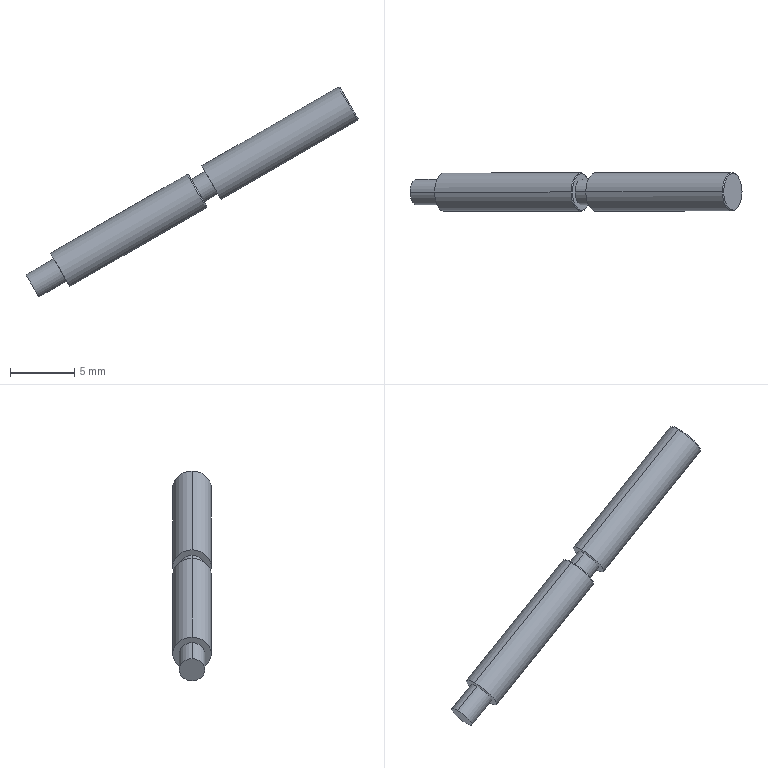Component | SolidWorks | SliderScrew1-1 | 1 solid | 17 faces | box 25.89 x 3 x 16.38 mm | volume 187 mm3 | cylinder 8 | plane 5 | cone 4 | commonest cylinder face diameters 2 x4 3 x4
build123d program:
from build123d import *

# Parameters (mm, degrees)
SKETCH1_R           = 1.5
BOSS_EXTRUDE1_DEPTH = 13
CHAMFER1_SIZE       = 0.08
SKETCH2_R           = 1.5
SKETCH2_R_2         = 1
CUT_EXTRUDE1_DEPTH  = 0.625
CHAMFER2_SIZE       = 0.08
BOSS_EXTRUDE2_START = 2.5
SKETCH3_R           = 1
BOSS_EXTRUDE2_DEPTH = 2.5


with BuildPart() as part:
    # Sketch1 → Boss-Extrude1 (new, symmetric)
    with BuildSketch(Plane(origin=(0, 0, 0), x_dir=(0, 0, -1), z_dir=(1, 0, 0))):
        with Locations(Location((0, 0, 0), (0, 0, 180))):
            Circle(SKETCH1_R)
    extrude(amount=BOSS_EXTRUDE1_DEPTH, both=True)

    # Chamfer1
    chamfer1_edges = [part.edges().sort_by_distance(p)[0] for p in [
        (13, 0, -1.5),
    ]]
    chamfer(chamfer1_edges, length=CHAMFER1_SIZE)

    # Sketch2 → Cut-Extrude1 (cut, symmetric)
    with BuildSketch(Plane(origin=(0, 0, 0), x_dir=(0, 0, -1), z_dir=(1, 0, 0))):
        with Locations(Location((0, 0, 0), (0, 0, 180))):
            Circle(SKETCH2_R)
        Circle(SKETCH2_R_2, mode=Mode.SUBTRACT)
    extrude(amount=CUT_EXTRUDE1_DEPTH, both=True, mode=Mode.SUBTRACT)

    # Chamfer2
    chamfer2_edges = [part.edges().sort_by_distance(p)[0] for p in [
        (-0.625, 0, -1.5),
    ]]
    chamfer(chamfer2_edges, length=CHAMFER2_SIZE)

    # Sketch3 → Boss-Extrude2 (add)
    with BuildSketch(Plane.ZY.offset(13).offset(BOSS_EXTRUDE2_START)):
        with Locations(Location((0, 0, 0), (0, 0, 180))):
            Circle(SKETCH3_R)
    extrude(amount=-BOSS_EXTRUDE2_DEPTH)


solid = part.part

# Placed as in the assembly
solid = solid.moved(Location((-69.691, 19.006, 123.217), (-94.246, 2.447, -29.909)))
STEP:
#1=CARTESIAN_POINT('',(-3.292,0.7483,4.58));
#2=VERTEX_POINT('',#1);
#3=CARTESIAN_POINT('',(-3.253,0.7483,4.512));
#4=VERTEX_POINT('',#3);
#5=CARTESIAN_POINT('',(-3.272,0.7483,4.546));
#6=DIRECTION('',(-0.866,0.,-0.5));
#7=DIRECTION('',(-0.5,-0.00000096,0.866));
#8=AXIS2_PLACEMENT_3D('',#5,#6,#7);
#9=CIRCLE('',#8,0.03937);
#10=EDGE_CURVE('',#2,#4,#9,.T.);
#11=ORIENTED_EDGE('',*,*,#10,.F.);
#12=CARTESIAN_POINT('',(-3.207,0.7483,4.629));
#13=VERTEX_POINT('',#12);
#14=CARTESIAN_POINT('',(-3.292,0.7483,4.58));
#15=DIRECTION('',(0.866,-0.,0.5));
#16=VECTOR('',#15,39.37);
#17=LINE('',#14,#16);
#18=EDGE_CURVE('',#2,#13,#17,.T.);
#19=ORIENTED_EDGE('',*,*,#18,.T.);
#20=CARTESIAN_POINT('',(-3.167,0.7483,4.561));
#21=VERTEX_POINT('',#20);
#22=CARTESIAN_POINT('',(-3.187,0.7483,4.595));
#23=DIRECTION('',(-0.866,0.,-0.5));
#24=DIRECTION('',(-0.5,-0.00000096,0.866));
#25=AXIS2_PLACEMENT_3D('',#22,#23,#24);
#26=CIRCLE('',#25,0.03937);
#27=EDGE_CURVE('',#13,#21,#26,.T.);
#28=ORIENTED_EDGE('',*,*,#27,.T.);
#29=CARTESIAN_POINT('',(-3.253,0.7483,4.512));
#30=DIRECTION('',(0.866,-0.,0.5));
#31=VECTOR('',#30,39.37);
#32=LINE('',#29,#31);
#33=EDGE_CURVE('',#4,#21,#32,.T.);
#34=ORIENTED_EDGE('',*,*,#33,.F.);
#35=EDGE_LOOP('',(#11,#19,#28,#34));
#36=FACE_OUTER_BOUND('',#35,.T.);
#37=CARTESIAN_POINT('',(-3.272,0.7483,4.546));
#38=DIRECTION('',(0.866,-0.,0.5));
#39=DIRECTION('',(0.5,0.00000096,-0.866));
#40=AXIS2_PLACEMENT_3D('',#37,#38,#39);
#41=CYLINDRICAL_SURFACE('',#40,0.03937);
#42=ADVANCED_FACE('',(#36),#41,.T.);
#43=CARTESIAN_POINT('',(-2.737,0.7483,4.79));
#44=VERTEX_POINT('',#43);
#45=CARTESIAN_POINT('',(-2.793,0.7483,4.887));
#46=VERTEX_POINT('',#45);
#47=CARTESIAN_POINT('',(-2.765,0.7483,4.839));
#48=DIRECTION('',(0.866,-0.,0.5));
#49=DIRECTION('',(0.5,0.00000096,-0.866));
#50=AXIS2_PLACEMENT_3D('',#47,#48,#49);
#51=CIRCLE('',#50,0.05591);
#52=EDGE_CURVE('',#44,#46,#51,.T.);
#53=ORIENTED_EDGE('',*,*,#52,.F.);
#54=CARTESIAN_POINT('',(-2.738,0.7483,4.786));
#55=VERTEX_POINT('',#54);
#56=CARTESIAN_POINT('',(-2.737,0.7483,4.79));
#57=DIRECTION('',(-0.2588,0.00000068,-0.9659));
#58=VECTOR('',#57,39.37);
#59=LINE('',#56,#58);
#60=EDGE_CURVE('',#44,#55,#59,.T.);
#61=ORIENTED_EDGE('',*,*,#60,.T.);
#62=CARTESIAN_POINT('',(-2.797,0.7483,4.888));
#63=VERTEX_POINT('',#62);
#64=CARTESIAN_POINT('',(-2.768,0.7483,4.837));
#65=DIRECTION('',(-0.866,0.,-0.5));
#66=DIRECTION('',(0.5,0.00000096,-0.866));
#67=AXIS2_PLACEMENT_3D('',#64,#65,#66);
#68=CIRCLE('',#67,0.05906);
#69=EDGE_CURVE('',#63,#55,#68,.T.);
#70=ORIENTED_EDGE('',*,*,#69,.F.);
#71=CARTESIAN_POINT('',(-2.793,0.7483,4.887));
#72=DIRECTION('',(-0.9659,-0.00000068,0.2588));
#73=VECTOR('',#72,39.37);
#74=LINE('',#71,#73);
#75=EDGE_CURVE('',#46,#63,#74,.T.);
#76=ORIENTED_EDGE('',*,*,#75,.F.);
#77=EDGE_LOOP('',(#53,#61,#70,#76));
#78=FACE_OUTER_BOUND('',#77,.T.);
#79=CARTESIAN_POINT('',(-2.765,0.7483,4.839));
#80=DIRECTION('',(-0.866,0.,-0.5));
#81=DIRECTION('',(-0.5,-0.00000096,0.866));
#82=AXIS2_PLACEMENT_3D('',#79,#80,#81);
#83=CONICAL_SURFACE('',#82,0.05591,0.7854);
#84=ADVANCED_FACE('',(#78),#83,.T.);
#85=ORIENTED_EDGE('',*,*,#69,.T.);
#86=CARTESIAN_POINT('',(-3.157,0.7483,4.544));
#87=VERTEX_POINT('',#86);
#88=CARTESIAN_POINT('',(-2.271,0.7483,5.056));
#89=DIRECTION('',(-0.866,0.,-0.5));
#90=VECTOR('',#89,39.37);
#91=LINE('',#88,#90);
#92=EDGE_CURVE('',#55,#87,#91,.T.);
#93=ORIENTED_EDGE('',*,*,#92,.T.);
#94=CARTESIAN_POINT('',(-3.217,0.7483,4.646));
#95=VERTEX_POINT('',#94);
#96=CARTESIAN_POINT('',(-3.187,0.7483,4.595));
#97=DIRECTION('',(0.866,-0.,0.5));
#98=DIRECTION('',(0.5,0.00000096,-0.866));
#99=AXIS2_PLACEMENT_3D('',#96,#97,#98);
#100=CIRCLE('',#99,0.05906);
#101=EDGE_CURVE('',#87,#95,#100,.T.);
#102=ORIENTED_EDGE('',*,*,#101,.T.);
#103=CARTESIAN_POINT('',(-2.33,0.7483,5.158));
#104=DIRECTION('',(-0.866,0.,-0.5));
#105=VECTOR('',#104,39.37);
#106=LINE('',#103,#105);
#107=EDGE_CURVE('',#63,#95,#106,.T.);
#108=ORIENTED_EDGE('',*,*,#107,.F.);
#109=EDGE_LOOP('',(#85,#93,#102,#108));
#110=FACE_OUTER_BOUND('',#109,.T.);
#111=CARTESIAN_POINT('',(-2.301,0.7483,5.107));
#112=DIRECTION('',(-0.866,0.,-0.5));
#113=DIRECTION('',(-0.5,-0.00000096,0.866));
#114=AXIS2_PLACEMENT_3D('',#111,#112,#113);
#115=CYLINDRICAL_SURFACE('',#114,0.05906);
#116=ADVANCED_FACE('',(#110),#115,.T.);
#117=CARTESIAN_POINT('',(-2.745,0.7483,4.805));
#118=VERTEX_POINT('',#117);
#119=CARTESIAN_POINT('',(-2.785,0.7483,4.873));
#120=VERTEX_POINT('',#119);
#121=CARTESIAN_POINT('',(-2.765,0.7483,4.839));
#122=DIRECTION('',(0.866,-0.,0.5));
#123=DIRECTION('',(0.5,0.00000096,-0.866));
#124=AXIS2_PLACEMENT_3D('',#121,#122,#123);
#125=CIRCLE('',#124,0.03937);
#126=EDGE_CURVE('',#118,#120,#125,.T.);
#127=ORIENTED_EDGE('',*,*,#126,.T.);
#128=CARTESIAN_POINT('',(-2.742,0.7483,4.897));
#129=VERTEX_POINT('',#128);
#130=CARTESIAN_POINT('',(-2.785,0.7483,4.873));
#131=DIRECTION('',(0.866,-0.,0.5));
#132=VECTOR('',#131,39.37);
#133=LINE('',#130,#132);
#134=EDGE_CURVE('',#120,#129,#133,.T.);
#135=ORIENTED_EDGE('',*,*,#134,.T.);
#136=CARTESIAN_POINT('',(-2.703,0.7483,4.829));
#137=VERTEX_POINT('',#136);
#138=CARTESIAN_POINT('',(-2.722,0.7483,4.863));
#139=DIRECTION('',(0.866,-0.,0.5));
#140=DIRECTION('',(0.5,0.00000096,-0.866));
#141=AXIS2_PLACEMENT_3D('',#138,#139,#140);
#142=CIRCLE('',#141,0.03937);
#143=EDGE_CURVE('',#137,#129,#142,.T.);
#144=ORIENTED_EDGE('',*,*,#143,.F.);
#145=CARTESIAN_POINT('',(-2.745,0.7483,4.805));
#146=DIRECTION('',(0.866,-0.,0.5));
#147=VECTOR('',#146,39.37);
#148=LINE('',#145,#147);
#149=EDGE_CURVE('',#118,#137,#148,.T.);
#150=ORIENTED_EDGE('',*,*,#149,.F.);
#151=EDGE_LOOP('',(#127,#135,#144,#150));
#152=FACE_OUTER_BOUND('',#151,.T.);
#153=CARTESIAN_POINT('',(-2.765,0.7483,4.839));
#154=DIRECTION('',(0.866,-0.,0.5));
#155=DIRECTION('',(0.5,0.00000096,-0.866));
#156=AXIS2_PLACEMENT_3D('',#153,#154,#155);
#157=CYLINDRICAL_SURFACE('',#156,0.03937);
#158=ADVANCED_FACE('',(#152),#157,.T.);
#159=CARTESIAN_POINT('',(-2.273,0.7483,5.059));
#160=VERTEX_POINT('',#159);
#161=CARTESIAN_POINT('',(-2.328,0.7483,5.155));
#162=VERTEX_POINT('',#161);
#163=CARTESIAN_POINT('',(-2.301,0.7483,5.107));
#164=DIRECTION('',(0.866,-0.,0.5));
#165=DIRECTION('',(0.5,0.00000096,-0.866));
#166=AXIS2_PLACEMENT_3D('',#163,#164,#165);
#167=CIRCLE('',#166,0.05591);
#168=EDGE_CURVE('',#160,#162,#167,.T.);
#169=ORIENTED_EDGE('',*,*,#168,.F.);
#170=CARTESIAN_POINT('',(-2.274,0.7483,5.054));
#171=VERTEX_POINT('',#170);
#172=CARTESIAN_POINT('',(-2.273,0.7483,5.059));
#173=DIRECTION('',(-0.2588,0.00000068,-0.9659));
#174=VECTOR('',#173,39.37);
#175=LINE('',#172,#174);
#176=EDGE_CURVE('',#160,#171,#175,.T.);
#177=ORIENTED_EDGE('',*,*,#176,.T.);
#178=CARTESIAN_POINT('',(-2.333,0.7483,5.157));
#179=VERTEX_POINT('',#178);
#180=CARTESIAN_POINT('',(-2.303,0.7483,5.105));
#181=DIRECTION('',(-0.866,0.,-0.5));
#182=DIRECTION('',(0.5,0.00000096,-0.866));
#183=AXIS2_PLACEMENT_3D('',#180,#181,#182);
#184=CIRCLE('',#183,0.05906);
#185=EDGE_CURVE('',#179,#171,#184,.T.);
#186=ORIENTED_EDGE('',*,*,#185,.F.);
#187=CARTESIAN_POINT('',(-2.328,0.7483,5.155));
#188=DIRECTION('',(-0.9659,-0.00000068,0.2588));
#189=VECTOR('',#188,39.37);
#190=LINE('',#187,#189);
#191=EDGE_CURVE('',#162,#179,#190,.T.);
#192=ORIENTED_EDGE('',*,*,#191,.F.);
#193=EDGE_LOOP('',(#169,#177,#186,#192));
#194=FACE_OUTER_BOUND('',#193,.T.);
#195=CARTESIAN_POINT('',(-2.301,0.7483,5.107));
#196=DIRECTION('',(-0.866,0.,-0.5));
#197=DIRECTION('',(-0.5,-0.00000096,0.866));
#198=AXIS2_PLACEMENT_3D('',#195,#196,#197);
#199=CONICAL_SURFACE('',#198,0.05591,0.7854);
#200=ADVANCED_FACE('',(#194),#199,.T.);
#201=ORIENTED_EDGE('',*,*,#185,.T.);
#202=CARTESIAN_POINT('',(-2.693,0.7483,4.812));
#203=VERTEX_POINT('',#202);
#204=CARTESIAN_POINT('',(-2.271,0.7483,5.056));
#205=DIRECTION('',(-0.866,0.,-0.5));
#206=VECTOR('',#205,39.37);
#207=LINE('',#204,#206);
#208=EDGE_CURVE('',#171,#203,#207,.T.);
#209=ORIENTED_EDGE('',*,*,#208,.T.);
#210=CARTESIAN_POINT('',(-2.752,0.7483,4.915));
#211=VERTEX_POINT('',#210);
#212=CARTESIAN_POINT('',(-2.722,0.7483,4.863));
#213=DIRECTION('',(0.866,-0.,0.5));
#214=DIRECTION('',(0.5,0.00000096,-0.866));
#215=AXIS2_PLACEMENT_3D('',#212,#213,#214);
#216=CIRCLE('',#215,0.05906);
#217=EDGE_CURVE('',#203,#211,#216,.T.);
#218=ORIENTED_EDGE('',*,*,#217,.T.);
#219=CARTESIAN_POINT('',(-2.33,0.7483,5.158));
#220=DIRECTION('',(-0.866,0.,-0.5));
#221=VECTOR('',#220,39.37);
#222=LINE('',#219,#221);
#223=EDGE_CURVE('',#179,#211,#222,.T.);
#224=ORIENTED_EDGE('',*,*,#223,.F.);
#225=EDGE_LOOP('',(#201,#209,#218,#224));
#226=FACE_OUTER_BOUND('',#225,.T.);
#227=CARTESIAN_POINT('',(-2.301,0.7483,5.107));
#228=DIRECTION('',(-0.866,0.,-0.5));
#229=DIRECTION('',(-0.5,-0.00000096,0.866));
#230=AXIS2_PLACEMENT_3D('',#227,#228,#229);
#231=CYLINDRICAL_SURFACE('',#230,0.05906);
#232=ADVANCED_FACE('',(#226),#231,.T.);
#233=ORIENTED_EDGE('',*,*,#208,.F.);
#234=CARTESIAN_POINT('',(-2.303,0.7483,5.105));
#235=DIRECTION('',(-0.866,0.,-0.5));
#236=DIRECTION('',(0.5,0.00000096,-0.866));
#237=AXIS2_PLACEMENT_3D('',#234,#235,#236);
#238=CIRCLE('',#237,0.05906);
#239=EDGE_CURVE('',#171,#179,#238,.T.);
#240=ORIENTED_EDGE('',*,*,#239,.T.);
#241=ORIENTED_EDGE('',*,*,#223,.T.);
#242=CARTESIAN_POINT('',(-2.722,0.7483,4.863));
#243=DIRECTION('',(0.866,-0.,0.5));
#244=DIRECTION('',(0.5,0.00000096,-0.866));
#245=AXIS2_PLACEMENT_3D('',#242,#243,#244);
#246=CIRCLE('',#245,0.05906);
#247=EDGE_CURVE('',#211,#203,#246,.T.);
#248=ORIENTED_EDGE('',*,*,#247,.T.);
#249=EDGE_LOOP('',(#233,#240,#241,#248));
#250=FACE_OUTER_BOUND('',#249,.T.);
#251=CARTESIAN_POINT('',(-2.301,0.7483,5.107));
#252=DIRECTION('',(-0.866,0.,-0.5));
#253=DIRECTION('',(-0.5,-0.00000096,0.866));
#254=AXIS2_PLACEMENT_3D('',#251,#252,#253);
#255=CYLINDRICAL_SURFACE('',#254,0.05906);
#256=ADVANCED_FACE('',(#250),#255,.T.);
#257=CARTESIAN_POINT('',(-2.301,0.7483,5.107));
#258=DIRECTION('',(0.866,-0.,0.5));
#259=DIRECTION('',(0.5,0.00000096,-0.866));
#260=AXIS2_PLACEMENT_3D('',#257,#258,#259);
#261=CIRCLE('',#260,0.05591);
#262=EDGE_CURVE('',#162,#160,#261,.T.);
#263=ORIENTED_EDGE('',*,*,#262,.T.);
#264=ORIENTED_EDGE('',*,*,#168,.T.);
#265=EDGE_LOOP('',(#263,#264));
#266=FACE_OUTER_BOUND('',#265,.T.);
#267=CARTESIAN_POINT('',(-2.301,0.7483,5.107));
#268=DIRECTION('',(0.866,-0.,0.5));
#269=DIRECTION('',(0.5,0.00000096,-0.866));
#270=AXIS2_PLACEMENT_3D('',#267,#268,#269);
#271=PLANE('',#270);
#272=ADVANCED_FACE('',(#266),#271,.T.);
#273=ORIENTED_EDGE('',*,*,#176,.F.);
#274=ORIENTED_EDGE('',*,*,#262,.F.);
#275=ORIENTED_EDGE('',*,*,#191,.T.);
#276=ORIENTED_EDGE('',*,*,#239,.F.);
#277=EDGE_LOOP('',(#273,#274,#275,#276));
#278=FACE_OUTER_BOUND('',#277,.T.);
#279=CARTESIAN_POINT('',(-2.301,0.7483,5.107));
#280=DIRECTION('',(-0.866,0.,-0.5));
#281=DIRECTION('',(-0.5,-0.00000096,0.866));
#282=AXIS2_PLACEMENT_3D('',#279,#280,#281);
#283=CONICAL_SURFACE('',#282,0.05591,0.7854);
#284=ADVANCED_FACE('',(#278),#283,.T.);
#285=CARTESIAN_POINT('',(-2.765,0.7483,4.839));
#286=DIRECTION('',(0.866,-0.,0.5));
#287=DIRECTION('',(0.5,0.00000096,-0.866));
#288=AXIS2_PLACEMENT_3D('',#285,#286,#287);
#289=CIRCLE('',#288,0.05591);
#290=EDGE_CURVE('',#46,#44,#289,.T.);
#291=ORIENTED_EDGE('',*,*,#290,.T.);
#292=ORIENTED_EDGE('',*,*,#52,.T.);
#293=EDGE_LOOP('',(#291,#292));
#294=FACE_OUTER_BOUND('',#293,.T.);
#295=ORIENTED_EDGE('',*,*,#126,.F.);
#296=CARTESIAN_POINT('',(-2.765,0.7483,4.839));
#297=DIRECTION('',(0.866,-0.,0.5));
#298=DIRECTION('',(0.5,0.00000096,-0.866));
#299=AXIS2_PLACEMENT_3D('',#296,#297,#298);
#300=CIRCLE('',#299,0.03937);
#301=EDGE_CURVE('',#120,#118,#300,.T.);
#302=ORIENTED_EDGE('',*,*,#301,.F.);
#303=EDGE_LOOP('',(#295,#302));
#304=FACE_BOUND('',#303,.T.);
#305=CARTESIAN_POINT('',(-2.765,0.7483,4.839));
#306=DIRECTION('',(0.866,-0.,0.5));
#307=DIRECTION('',(0.5,0.00000096,-0.866));
#308=AXIS2_PLACEMENT_3D('',#305,#306,#307);
#309=PLANE('',#308);
#310=ADVANCED_FACE('',(#294,#304),#309,.T.);
#311=ORIENTED_EDGE('',*,*,#143,.T.);
#312=CARTESIAN_POINT('',(-2.722,0.7483,4.863));
#313=DIRECTION('',(0.866,-0.,0.5));
#314=DIRECTION('',(0.5,0.00000096,-0.866));
#315=AXIS2_PLACEMENT_3D('',#312,#313,#314);
#316=CIRCLE('',#315,0.03937);
#317=EDGE_CURVE('',#129,#137,#316,.T.);
#318=ORIENTED_EDGE('',*,*,#317,.T.);
#319=EDGE_LOOP('',(#311,#318));
#320=FACE_BOUND('',#319,.T.);
#321=ORIENTED_EDGE('',*,*,#247,.F.);
#322=ORIENTED_EDGE('',*,*,#217,.F.);
#323=EDGE_LOOP('',(#321,#322));
#324=FACE_OUTER_BOUND('',#323,.T.);
#325=CARTESIAN_POINT('',(-2.722,0.7483,4.863));
#326=DIRECTION('',(0.866,-0.,0.5));
#327=DIRECTION('',(0.5,0.00000096,-0.866));
#328=AXIS2_PLACEMENT_3D('',#325,#326,#327);
#329=PLANE('',#328);
#330=ADVANCED_FACE('',(#320,#324),#329,.F.);
#331=ORIENTED_EDGE('',*,*,#134,.F.);
#332=ORIENTED_EDGE('',*,*,#301,.T.);
#333=ORIENTED_EDGE('',*,*,#149,.T.);
#334=ORIENTED_EDGE('',*,*,#317,.F.);
#335=EDGE_LOOP('',(#331,#332,#333,#334));
#336=FACE_OUTER_BOUND('',#335,.T.);
#337=CARTESIAN_POINT('',(-2.765,0.7483,4.839));
#338=DIRECTION('',(0.866,-0.,0.5));
#339=DIRECTION('',(0.5,0.00000096,-0.866));
#340=AXIS2_PLACEMENT_3D('',#337,#338,#339);
#341=CYLINDRICAL_SURFACE('',#340,0.03937);
#342=ADVANCED_FACE('',(#336),#341,.T.);
#343=CARTESIAN_POINT('',(-3.187,0.7483,4.595));
#344=DIRECTION('',(-0.866,0.,-0.5));
#345=DIRECTION('',(-0.5,-0.00000096,0.866));
#346=AXIS2_PLACEMENT_3D('',#343,#344,#345);
#347=CIRCLE('',#346,0.03937);
#348=EDGE_CURVE('',#21,#13,#347,.T.);
#349=ORIENTED_EDGE('',*,*,#348,.F.);
#350=ORIENTED_EDGE('',*,*,#27,.F.);
#351=EDGE_LOOP('',(#349,#350));
#352=FACE_BOUND('',#351,.T.);
#353=CARTESIAN_POINT('',(-3.187,0.7483,4.595));
#354=DIRECTION('',(0.866,-0.,0.5));
#355=DIRECTION('',(0.5,0.00000096,-0.866));
#356=AXIS2_PLACEMENT_3D('',#353,#354,#355);
#357=CIRCLE('',#356,0.05906);
#358=EDGE_CURVE('',#95,#87,#357,.T.);
#359=ORIENTED_EDGE('',*,*,#358,.F.);
#360=ORIENTED_EDGE('',*,*,#101,.F.);
#361=EDGE_LOOP('',(#359,#360));
#362=FACE_OUTER_BOUND('',#361,.T.);
#363=CARTESIAN_POINT('',(-3.187,0.7483,4.595));
#364=DIRECTION('',(0.866,-0.,0.5));
#365=DIRECTION('',(0.5,0.00000096,-0.866));
#366=AXIS2_PLACEMENT_3D('',#363,#364,#365);
#367=PLANE('',#366);
#368=ADVANCED_FACE('',(#352,#362),#367,.F.);
#369=ORIENTED_EDGE('',*,*,#92,.F.);
#370=CARTESIAN_POINT('',(-2.768,0.7483,4.837));
#371=DIRECTION('',(-0.866,0.,-0.5));
#372=DIRECTION('',(0.5,0.00000096,-0.866));
#373=AXIS2_PLACEMENT_3D('',#370,#371,#372);
#374=CIRCLE('',#373,0.05906);
#375=EDGE_CURVE('',#55,#63,#374,.T.);
#376=ORIENTED_EDGE('',*,*,#375,.T.);
#377=ORIENTED_EDGE('',*,*,#107,.T.);
#378=ORIENTED_EDGE('',*,*,#358,.T.);
#379=EDGE_LOOP('',(#369,#376,#377,#378));
#380=FACE_OUTER_BOUND('',#379,.T.);
#381=CARTESIAN_POINT('',(-2.301,0.7483,5.107));
#382=DIRECTION('',(-0.866,0.,-0.5));
#383=DIRECTION('',(-0.5,-0.00000096,0.866));
#384=AXIS2_PLACEMENT_3D('',#381,#382,#383);
#385=CYLINDRICAL_SURFACE('',#384,0.05906);
#386=ADVANCED_FACE('',(#380),#385,.T.);
#387=ORIENTED_EDGE('',*,*,#60,.F.);
#388=ORIENTED_EDGE('',*,*,#290,.F.);
#389=ORIENTED_EDGE('',*,*,#75,.T.);
#390=ORIENTED_EDGE('',*,*,#375,.F.);
#391=EDGE_LOOP('',(#387,#388,#389,#390));
#392=FACE_OUTER_BOUND('',#391,.T.);
#393=CARTESIAN_POINT('',(-2.765,0.7483,4.839));
#394=DIRECTION('',(-0.866,0.,-0.5));
#395=DIRECTION('',(-0.5,-0.00000096,0.866));
#396=AXIS2_PLACEMENT_3D('',#393,#394,#395);
#397=CONICAL_SURFACE('',#396,0.05591,0.7854);
#398=ADVANCED_FACE('',(#392),#397,.T.);
#399=ORIENTED_EDGE('',*,*,#18,.F.);
#400=CARTESIAN_POINT('',(-3.272,0.7483,4.546));
#401=DIRECTION('',(-0.866,0.,-0.5));
#402=DIRECTION('',(-0.5,-0.00000096,0.866));
#403=AXIS2_PLACEMENT_3D('',#400,#401,#402);
#404=CIRCLE('',#403,0.03937);
#405=EDGE_CURVE('',#4,#2,#404,.T.);
#406=ORIENTED_EDGE('',*,*,#405,.F.);
#407=ORIENTED_EDGE('',*,*,#33,.T.);
#408=ORIENTED_EDGE('',*,*,#348,.T.);
#409=EDGE_LOOP('',(#399,#406,#407,#408));
#410=FACE_OUTER_BOUND('',#409,.T.);
#411=CARTESIAN_POINT('',(-3.272,0.7483,4.546));
#412=DIRECTION('',(0.866,-0.,0.5));
#413=DIRECTION('',(0.5,0.00000096,-0.866));
#414=AXIS2_PLACEMENT_3D('',#411,#412,#413);
#415=CYLINDRICAL_SURFACE('',#414,0.03937);
#416=ADVANCED_FACE('',(#410),#415,.T.);
#417=ORIENTED_EDGE('',*,*,#405,.T.);
#418=ORIENTED_EDGE('',*,*,#10,.T.);
#419=EDGE_LOOP('',(#417,#418));
#420=FACE_OUTER_BOUND('',#419,.T.);
#421=CARTESIAN_POINT('',(-3.272,0.7483,4.546));
#422=DIRECTION('',(-0.866,0.,-0.5));
#423=DIRECTION('',(-0.5,-0.00000096,0.866));
#424=AXIS2_PLACEMENT_3D('',#421,#422,#423);
#425=PLANE('',#424);
#426=ADVANCED_FACE('',(#420),#425,.T.);
#427=CLOSED_SHELL('',(#42,#84,#116,#158,#200,#232,#256,#272,#284,#310,#330,#342,#368,#386,#398,#416,#426));
#428=MANIFOLD_SOLID_BREP('',#427);
#429=CARTESIAN_POINT('',(0.,0.,0.));
#430=DIRECTION('',(0.,0.,1.));
#431=DIRECTION('',(1.,0.,0.));
#432=AXIS2_PLACEMENT_3D('',#429,#430,#431);
#433=(LENGTH_UNIT()NAMED_UNIT(*)SI_UNIT($,.METRE.));
#434=LENGTH_MEASURE_WITH_UNIT(LENGTH_MEASURE(0.0254),#433);
#435=DIMENSIONAL_EXPONENTS(1.,0.,0.,0.,0.,0.,0.);
#436=(CONVERSION_BASED_UNIT('',#434)LENGTH_UNIT()NAMED_UNIT(#435));
#437=UNCERTAINTY_MEASURE_WITH_UNIT(LENGTH_MEASURE(0.00001),#436,'','');
#438=(NAMED_UNIT(*)PLANE_ANGLE_UNIT()SI_UNIT($,.RADIAN.));
#439=(NAMED_UNIT(*)SI_UNIT($,.STERADIAN.)SOLID_ANGLE_UNIT());
#440=(GEOMETRIC_REPRESENTATION_CONTEXT(3)GLOBAL_UNCERTAINTY_ASSIGNED_CONTEXT((#437))GLOBAL_UNIT_ASSIGNED_CONTEXT((#436,#438,#439))REPRESENTATION_CONTEXT('',''));
#441=ADVANCED_BREP_SHAPE_REPRESENTATION('',(#428,#432),#440);
#442=COLOUR_RGB('',0.7922,0.8196,0.9333);
#443=FILL_AREA_STYLE_COLOUR('',#442);
#444=FILL_AREA_STYLE('',(#443));
#445=SURFACE_STYLE_FILL_AREA(#444);
#446=SURFACE_SIDE_STYLE('',(#445));
#447=SURFACE_STYLE_USAGE(.BOTH.,#446);
#448=PRESENTATION_STYLE_ASSIGNMENT((#447));
#449=STYLED_ITEM('',(#448),#428);
#450=(LENGTH_UNIT()NAMED_UNIT(*)SI_UNIT($,.METRE.));
#451=LENGTH_MEASURE_WITH_UNIT(LENGTH_MEASURE(0.0254),#450);
#452=DIMENSIONAL_EXPONENTS(1.,0.,0.,0.,0.,0.,0.);
#453=(CONVERSION_BASED_UNIT('',#451)LENGTH_UNIT()NAMED_UNIT(#452));
#454=UNCERTAINTY_MEASURE_WITH_UNIT(LENGTH_MEASURE(0.00001),#453,'','');
#455=(NAMED_UNIT(*)PLANE_ANGLE_UNIT()SI_UNIT($,.RADIAN.));
#456=(NAMED_UNIT(*)SI_UNIT($,.STERADIAN.)SOLID_ANGLE_UNIT());
#457=(GEOMETRIC_REPRESENTATION_CONTEXT(3)GLOBAL_UNCERTAINTY_ASSIGNED_CONTEXT((#454))GLOBAL_UNIT_ASSIGNED_CONTEXT((#453,#455,#456))REPRESENTATION_CONTEXT('',''));
#458=MECHANICAL_DESIGN_GEOMETRIC_PRESENTATION_REPRESENTATION('',(#449),#457);
#459=PRESENTATION_LAYER_ASSIGNMENT('','',(#449));